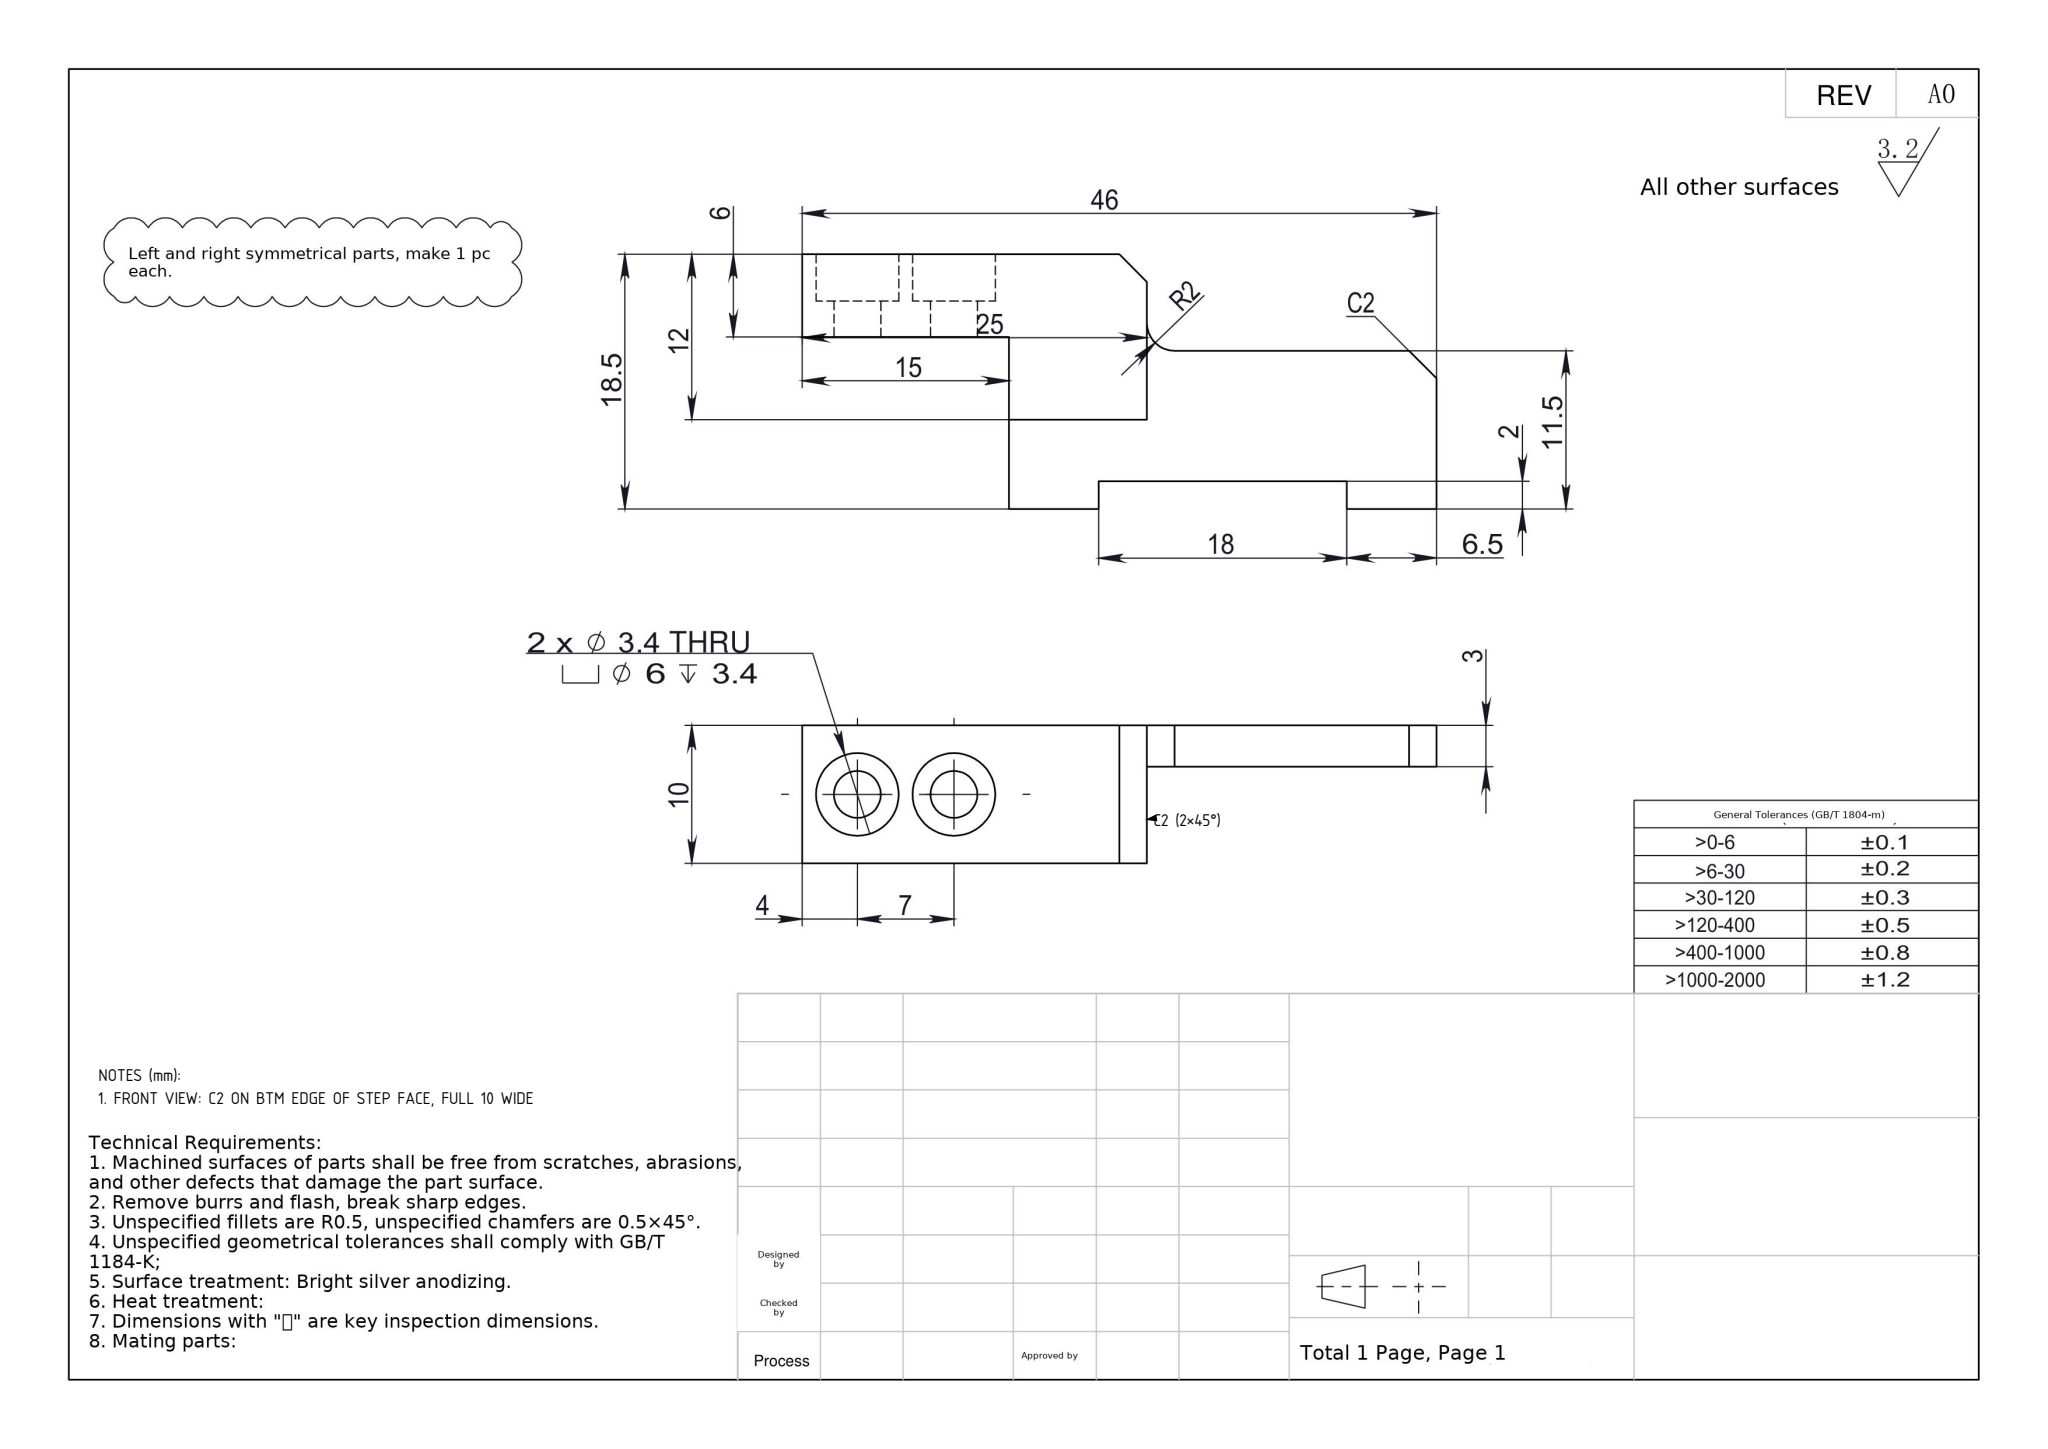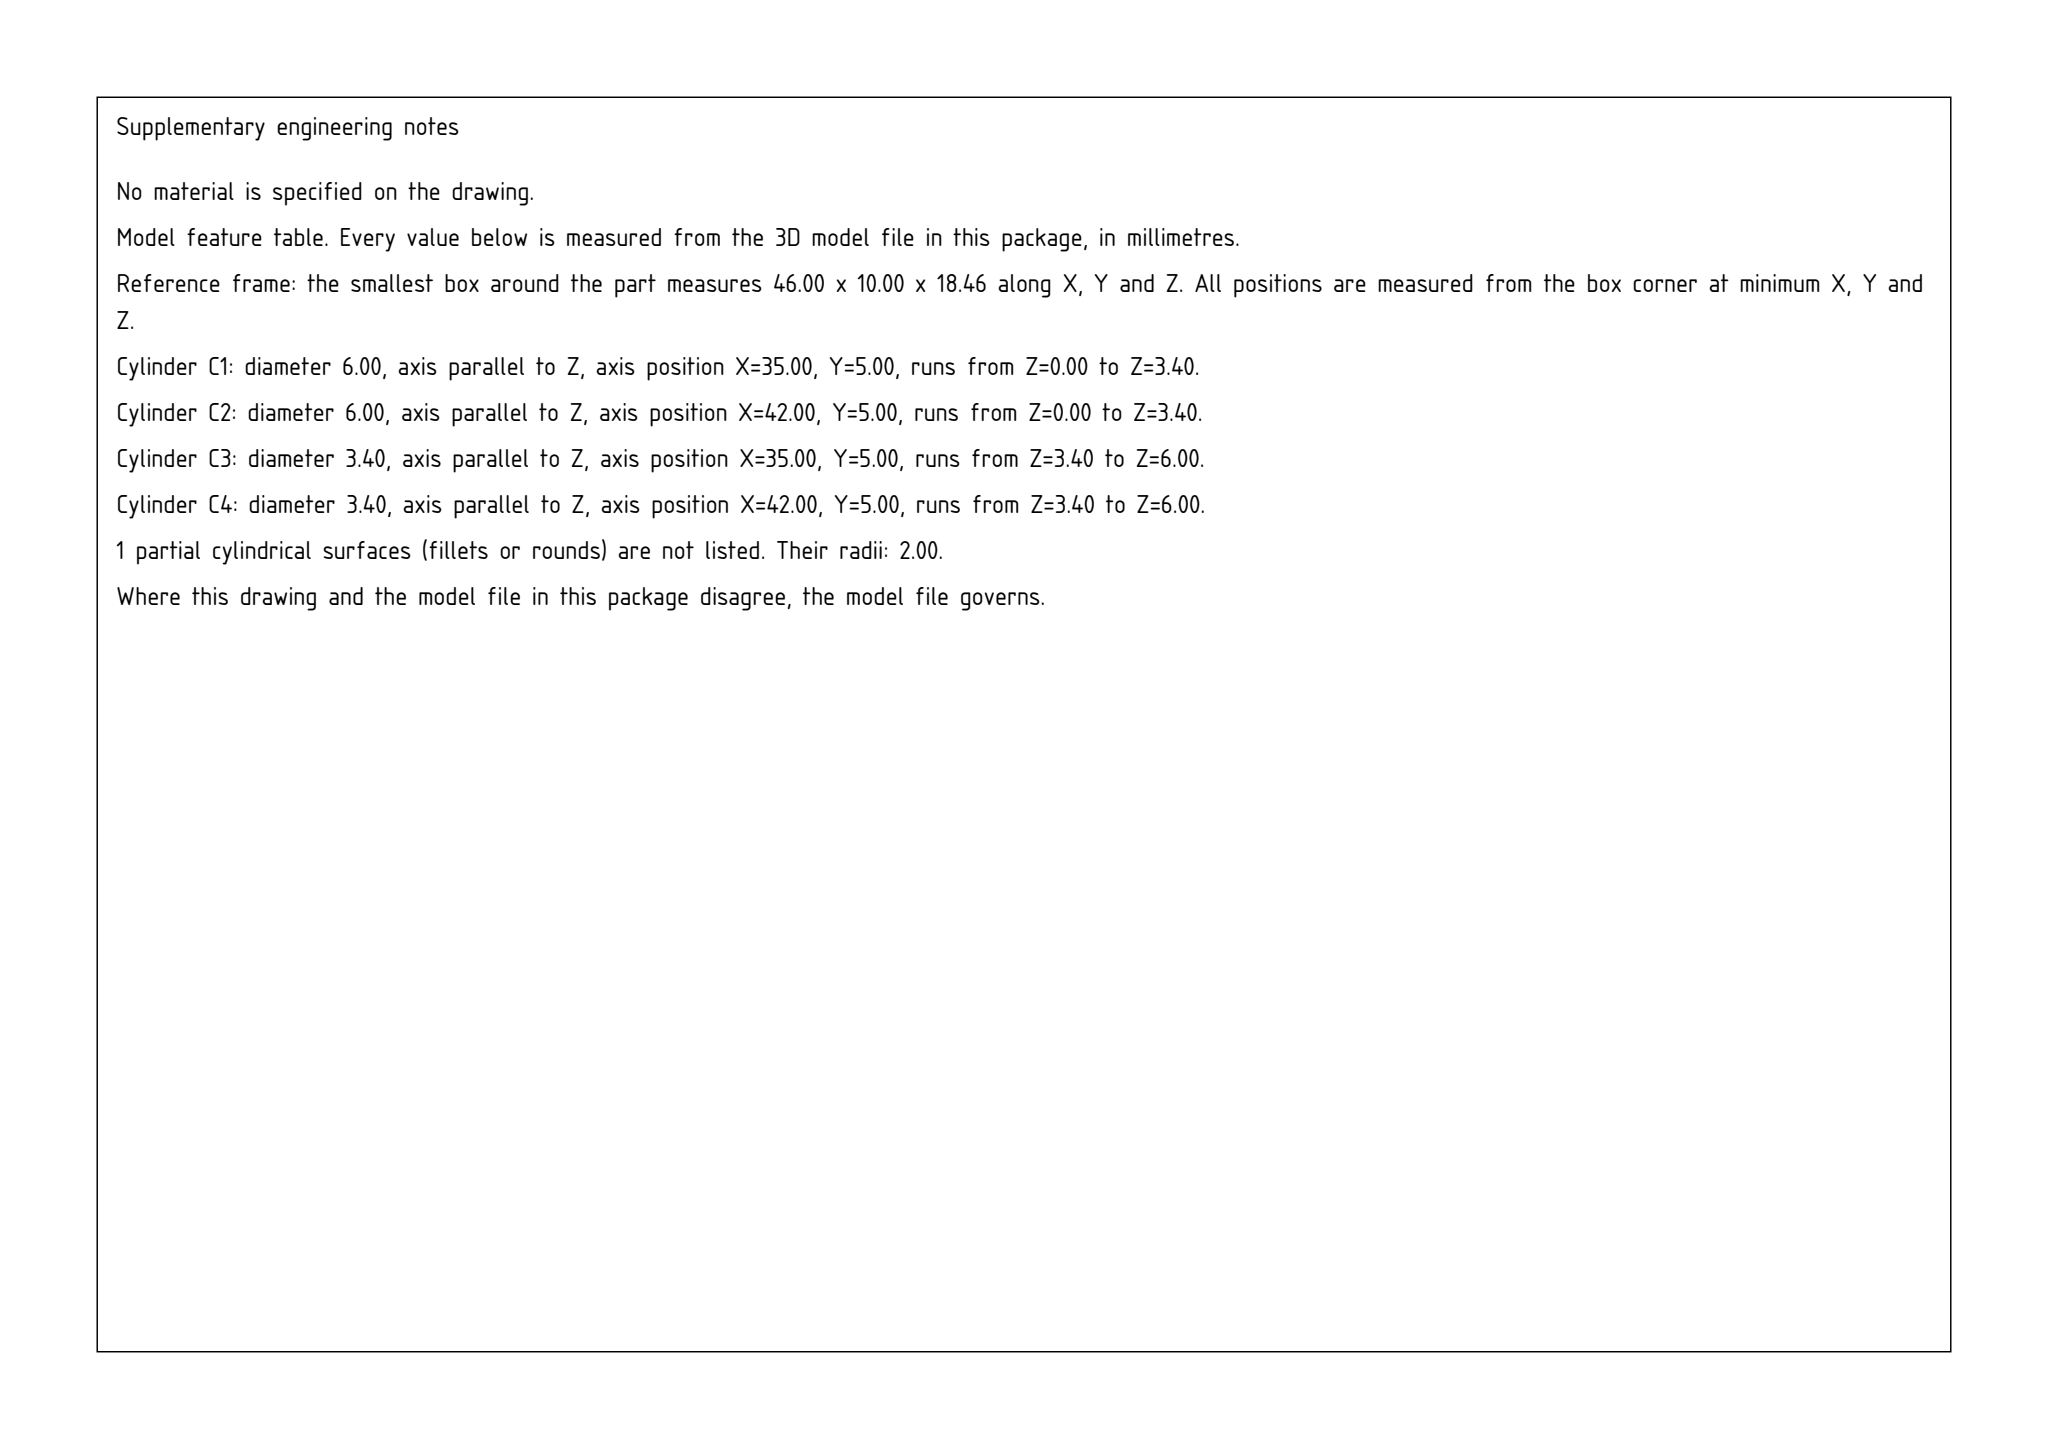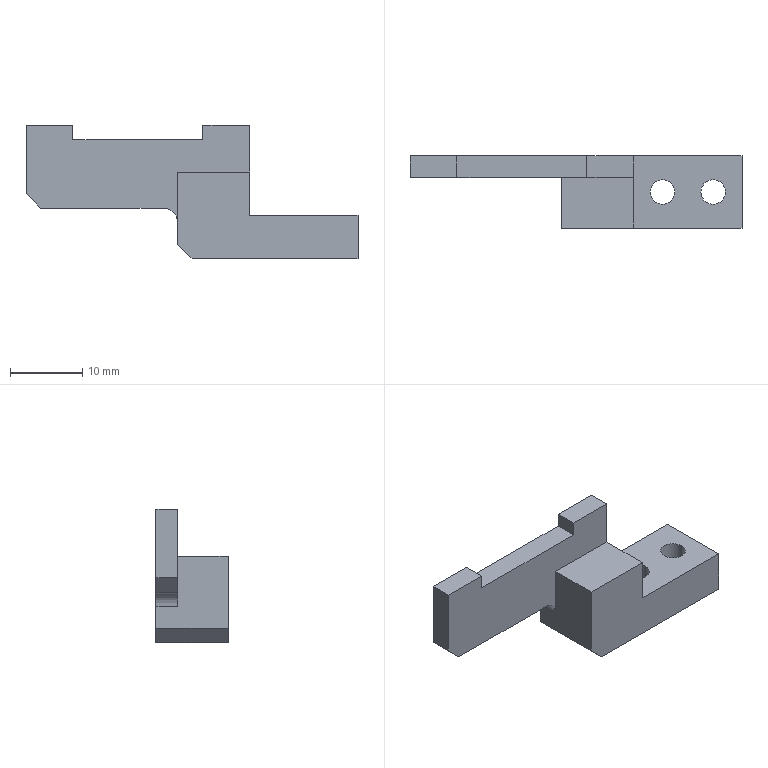Part | SolidWorks | mm | 1 solid | 29 faces | box 46 x 10 x 18.46 mm | volume 2645 mm3 | plane 20 | cylinder 9 | commonest cylinder face diameters 6 x4 3.4 x4 4 x1
Drawing notes:
FRONT VIEW: C2 ON BTM EDGE OF STEP FACE, FULL 10 WIDE | from the solid: inclined plane 45°, bbox_from [21,0,0], size [2,10,2] joining z=0 face and x=21 step face
FRONT VIEW: C2 (2x45 DEG) AT BOTTOM EDGE OF 18 STEP WALL | from the solid: inclined_plane 45/90/45 at bbox_from [21,0,0], size [2,10,2]: 2x2 chamfer between z=0 face (x 23-46) and x=21 face (z from 2)
STEP:
#1=CARTESIAN_POINT('',(-13.,5.,-18.6));
#2=VERTEX_POINT('',#1);
#3=CARTESIAN_POINT('',(-19.,5.,-18.6));
#4=VERTEX_POINT('',#3);
#5=CARTESIAN_POINT('',(-16.,5.,-18.6));
#6=DIRECTION('',(0.,0.,-1.));
#7=DIRECTION('',(-1.,0.,0.));
#8=AXIS2_PLACEMENT_3D('',#5,#6,#7);
#9=CIRCLE('',#8,3.);
#10=EDGE_CURVE('',#2,#4,#9,.T.);
#11=ORIENTED_EDGE('',*,*,#10,.F.);
#12=CARTESIAN_POINT('',(-13.,5.,-22.));
#13=VERTEX_POINT('',#12);
#14=CARTESIAN_POINT('',(-13.,5.,-22.));
#15=DIRECTION('',(0.,0.,-1.));
#16=VECTOR('',#15,1000.);
#17=LINE('',#14,#16);
#18=EDGE_CURVE('',#2,#13,#17,.T.);
#19=ORIENTED_EDGE('',*,*,#18,.T.);
#20=CARTESIAN_POINT('',(-19.,5.,-22.));
#21=VERTEX_POINT('',#20);
#22=CARTESIAN_POINT('',(-16.,5.,-22.));
#23=DIRECTION('',(0.,0.,-1.));
#24=DIRECTION('',(-1.,0.,0.));
#25=AXIS2_PLACEMENT_3D('',#22,#23,#24);
#26=CIRCLE('',#25,3.);
#27=EDGE_CURVE('',#13,#21,#26,.T.);
#28=ORIENTED_EDGE('',*,*,#27,.T.);
#29=CARTESIAN_POINT('',(-19.,5.,-22.));
#30=DIRECTION('',(0.,0.,-1.));
#31=VECTOR('',#30,1000.);
#32=LINE('',#29,#31);
#33=EDGE_CURVE('',#4,#21,#32,.T.);
#34=ORIENTED_EDGE('',*,*,#33,.F.);
#35=EDGE_LOOP('',(#11,#19,#28,#34));
#36=FACE_OUTER_BOUND('',#35,.T.);
#37=CARTESIAN_POINT('',(-16.,5.,-22.));
#38=DIRECTION('',(0.,0.,-1.));
#39=DIRECTION('',(-1.,0.,0.));
#40=AXIS2_PLACEMENT_3D('',#37,#38,#39);
#41=CYLINDRICAL_SURFACE('',#40,3.);
#42=ADVANCED_FACE('',(#36),#41,.F.);
#43=CARTESIAN_POINT('',(-14.3,5.,-16.));
#44=VERTEX_POINT('',#43);
#45=CARTESIAN_POINT('',(-17.7,5.,-16.));
#46=VERTEX_POINT('',#45);
#47=CARTESIAN_POINT('',(-16.,5.,-16.));
#48=DIRECTION('',(-0.,0.,-1.));
#49=DIRECTION('',(-1.,0.,0.));
#50=AXIS2_PLACEMENT_3D('',#47,#48,#49);
#51=CIRCLE('',#50,1.7);
#52=EDGE_CURVE('',#44,#46,#51,.T.);
#53=ORIENTED_EDGE('',*,*,#52,.F.);
#54=CARTESIAN_POINT('',(-14.3,5.,-18.6));
#55=VERTEX_POINT('',#54);
#56=CARTESIAN_POINT('',(-14.3,5.,-22.));
#57=DIRECTION('',(0.,0.,-1.));
#58=VECTOR('',#57,1000.);
#59=LINE('',#56,#58);
#60=EDGE_CURVE('',#44,#55,#59,.T.);
#61=ORIENTED_EDGE('',*,*,#60,.T.);
#62=CARTESIAN_POINT('',(-17.7,5.,-18.6));
#63=VERTEX_POINT('',#62);
#64=CARTESIAN_POINT('',(-16.,5.,-18.6));
#65=DIRECTION('',(0.,0.,-1.));
#66=DIRECTION('',(-1.,0.,0.));
#67=AXIS2_PLACEMENT_3D('',#64,#65,#66);
#68=CIRCLE('',#67,1.7);
#69=EDGE_CURVE('',#55,#63,#68,.T.);
#70=ORIENTED_EDGE('',*,*,#69,.T.);
#71=CARTESIAN_POINT('',(-17.7,5.,-22.));
#72=DIRECTION('',(0.,0.,-1.));
#73=VECTOR('',#72,1000.);
#74=LINE('',#71,#73);
#75=EDGE_CURVE('',#46,#63,#74,.T.);
#76=ORIENTED_EDGE('',*,*,#75,.F.);
#77=EDGE_LOOP('',(#53,#61,#70,#76));
#78=FACE_OUTER_BOUND('',#77,.T.);
#79=CARTESIAN_POINT('',(-16.,5.,-22.));
#80=DIRECTION('',(0.,0.,-1.));
#81=DIRECTION('',(-1.,0.,0.));
#82=AXIS2_PLACEMENT_3D('',#79,#80,#81);
#83=CYLINDRICAL_SURFACE('',#82,1.7);
#84=ADVANCED_FACE('',(#78),#83,.F.);
#85=CARTESIAN_POINT('',(-6.,5.,-18.6));
#86=VERTEX_POINT('',#85);
#87=CARTESIAN_POINT('',(-12.,5.,-18.6));
#88=VERTEX_POINT('',#87);
#89=CARTESIAN_POINT('',(-9.,5.,-18.6));
#90=DIRECTION('',(0.,0.,-1.));
#91=DIRECTION('',(-1.,0.,0.));
#92=AXIS2_PLACEMENT_3D('',#89,#90,#91);
#93=CIRCLE('',#92,3.);
#94=EDGE_CURVE('',#86,#88,#93,.T.);
#95=ORIENTED_EDGE('',*,*,#94,.F.);
#96=CARTESIAN_POINT('',(-6.,5.,-22.));
#97=VERTEX_POINT('',#96);
#98=CARTESIAN_POINT('',(-6.,5.,-22.));
#99=DIRECTION('',(0.,0.,-1.));
#100=VECTOR('',#99,1000.);
#101=LINE('',#98,#100);
#102=EDGE_CURVE('',#86,#97,#101,.T.);
#103=ORIENTED_EDGE('',*,*,#102,.T.);
#104=CARTESIAN_POINT('',(-12.,5.,-22.));
#105=VERTEX_POINT('',#104);
#106=CARTESIAN_POINT('',(-9.,5.,-22.));
#107=DIRECTION('',(0.,0.,-1.));
#108=DIRECTION('',(-1.,0.,0.));
#109=AXIS2_PLACEMENT_3D('',#106,#107,#108);
#110=CIRCLE('',#109,3.);
#111=EDGE_CURVE('',#97,#105,#110,.T.);
#112=ORIENTED_EDGE('',*,*,#111,.T.);
#113=CARTESIAN_POINT('',(-12.,5.,-22.));
#114=DIRECTION('',(0.,0.,-1.));
#115=VECTOR('',#114,1000.);
#116=LINE('',#113,#115);
#117=EDGE_CURVE('',#88,#105,#116,.T.);
#118=ORIENTED_EDGE('',*,*,#117,.F.);
#119=EDGE_LOOP('',(#95,#103,#112,#118));
#120=FACE_OUTER_BOUND('',#119,.T.);
#121=CARTESIAN_POINT('',(-9.,5.,-22.));
#122=DIRECTION('',(0.,0.,-1.));
#123=DIRECTION('',(-1.,0.,0.));
#124=AXIS2_PLACEMENT_3D('',#121,#122,#123);
#125=CYLINDRICAL_SURFACE('',#124,3.);
#126=ADVANCED_FACE('',(#120),#125,.F.);
#127=CARTESIAN_POINT('',(-7.3,5.,-16.));
#128=VERTEX_POINT('',#127);
#129=CARTESIAN_POINT('',(-10.7,5.,-16.));
#130=VERTEX_POINT('',#129);
#131=CARTESIAN_POINT('',(-9.,5.,-16.));
#132=DIRECTION('',(-0.,0.,-1.));
#133=DIRECTION('',(-1.,0.,0.));
#134=AXIS2_PLACEMENT_3D('',#131,#132,#133);
#135=CIRCLE('',#134,1.7);
#136=EDGE_CURVE('',#128,#130,#135,.T.);
#137=ORIENTED_EDGE('',*,*,#136,.F.);
#138=CARTESIAN_POINT('',(-7.3,5.,-18.6));
#139=VERTEX_POINT('',#138);
#140=CARTESIAN_POINT('',(-7.3,5.,-22.));
#141=DIRECTION('',(0.,0.,-1.));
#142=VECTOR('',#141,1000.);
#143=LINE('',#140,#142);
#144=EDGE_CURVE('',#128,#139,#143,.T.);
#145=ORIENTED_EDGE('',*,*,#144,.T.);
#146=CARTESIAN_POINT('',(-10.7,5.,-18.6));
#147=VERTEX_POINT('',#146);
#148=CARTESIAN_POINT('',(-9.,5.,-18.6));
#149=DIRECTION('',(0.,0.,-1.));
#150=DIRECTION('',(-1.,0.,0.));
#151=AXIS2_PLACEMENT_3D('',#148,#149,#150);
#152=CIRCLE('',#151,1.7);
#153=EDGE_CURVE('',#139,#147,#152,.T.);
#154=ORIENTED_EDGE('',*,*,#153,.T.);
#155=CARTESIAN_POINT('',(-10.7,5.,-22.));
#156=DIRECTION('',(0.,0.,-1.));
#157=VECTOR('',#156,1000.);
#158=LINE('',#155,#157);
#159=EDGE_CURVE('',#130,#147,#158,.T.);
#160=ORIENTED_EDGE('',*,*,#159,.F.);
#161=EDGE_LOOP('',(#137,#145,#154,#160));
#162=FACE_OUTER_BOUND('',#161,.T.);
#163=CARTESIAN_POINT('',(-9.,5.,-22.));
#164=DIRECTION('',(0.,0.,-1.));
#165=DIRECTION('',(-1.,0.,0.));
#166=AXIS2_PLACEMENT_3D('',#163,#164,#165);
#167=CYLINDRICAL_SURFACE('',#166,1.7);
#168=ADVANCED_FACE('',(#162),#167,.F.);
#169=CARTESIAN_POINT('',(-44.5,7.,-3.54));
#170=VERTEX_POINT('',#169);
#171=CARTESIAN_POINT('',(-51.,7.,-3.54));
#172=VERTEX_POINT('',#171);
#173=CARTESIAN_POINT('',(-30.,7.,-3.54));
#174=DIRECTION('',(-1.,0.,0.));
#175=VECTOR('',#174,1000.);
#176=LINE('',#173,#175);
#177=EDGE_CURVE('',#170,#172,#176,.T.);
#178=ORIENTED_EDGE('',*,*,#177,.F.);
#179=CARTESIAN_POINT('',(-44.5,10.,-3.54));
#180=VERTEX_POINT('',#179);
#181=CARTESIAN_POINT('',(-44.5,0.,-3.54));
#182=DIRECTION('',(0.,1.,0.));
#183=VECTOR('',#182,1000.);
#184=LINE('',#181,#183);
#185=EDGE_CURVE('',#170,#180,#184,.T.);
#186=ORIENTED_EDGE('',*,*,#185,.T.);
#187=CARTESIAN_POINT('',(-51.,10.,-3.54));
#188=VERTEX_POINT('',#187);
#189=CARTESIAN_POINT('',(-51.762,10.,-3.54));
#190=DIRECTION('',(-1.,0.,0.));
#191=VECTOR('',#190,1000.);
#192=LINE('',#189,#191);
#193=EDGE_CURVE('',#180,#188,#192,.T.);
#194=ORIENTED_EDGE('',*,*,#193,.T.);
#195=CARTESIAN_POINT('',(-51.,10.,-3.54));
#196=DIRECTION('',(0.,1.,0.));
#197=VECTOR('',#196,1000.);
#198=LINE('',#195,#197);
#199=EDGE_CURVE('',#172,#188,#198,.T.);
#200=ORIENTED_EDGE('',*,*,#199,.F.);
#201=EDGE_LOOP('',(#178,#186,#194,#200));
#202=FACE_OUTER_BOUND('',#201,.T.);
#203=CARTESIAN_POINT('',(-51.762,0.,-3.54));
#204=DIRECTION('',(0.,0.,-1.));
#205=DIRECTION('',(-1.,0.,0.));
#206=AXIS2_PLACEMENT_3D('',#203,#204,#205);
#207=PLANE('',#206);
#208=ADVANCED_FACE('',(#202),#207,.F.);
#209=CARTESIAN_POINT('',(-30.,7.,-17.));
#210=VERTEX_POINT('',#209);
#211=CARTESIAN_POINT('',(-30.,7.,-10.));
#212=VERTEX_POINT('',#211);
#213=CARTESIAN_POINT('',(-30.,7.,-15.));
#214=DIRECTION('',(0.,0.,1.));
#215=VECTOR('',#214,1000.);
#216=LINE('',#213,#215);
#217=EDGE_CURVE('',#210,#212,#216,.T.);
#218=ORIENTED_EDGE('',*,*,#217,.F.);
#219=CARTESIAN_POINT('',(-30.,10.,-17.));
#220=VERTEX_POINT('',#219);
#221=CARTESIAN_POINT('',(-30.,0.,-17.));
#222=DIRECTION('',(0.,1.,0.));
#223=VECTOR('',#222,1000.);
#224=LINE('',#221,#223);
#225=EDGE_CURVE('',#210,#220,#224,.T.);
#226=ORIENTED_EDGE('',*,*,#225,.T.);
#227=CARTESIAN_POINT('',(-30.,10.,-20.));
#228=VERTEX_POINT('',#227);
#229=CARTESIAN_POINT('',(-30.,10.,-22.));
#230=DIRECTION('',(0.,0.,-1.));
#231=VECTOR('',#230,1000.);
#232=LINE('',#229,#231);
#233=EDGE_CURVE('',#220,#228,#232,.T.);
#234=ORIENTED_EDGE('',*,*,#233,.T.);
#235=CARTESIAN_POINT('',(-30.,0.,-20.));
#236=VERTEX_POINT('',#235);
#237=CARTESIAN_POINT('',(-30.,0.,-20.));
#238=DIRECTION('',(0.,-1.,0.));
#239=VECTOR('',#238,1000.);
#240=LINE('',#237,#239);
#241=EDGE_CURVE('',#228,#236,#240,.T.);
#242=ORIENTED_EDGE('',*,*,#241,.T.);
#243=CARTESIAN_POINT('',(-30.,0.,-10.));
#244=VERTEX_POINT('',#243);
#245=CARTESIAN_POINT('',(-30.,0.,-22.));
#246=DIRECTION('',(0.,0.,-1.));
#247=VECTOR('',#246,1000.);
#248=LINE('',#245,#247);
#249=EDGE_CURVE('',#244,#236,#248,.T.);
#250=ORIENTED_EDGE('',*,*,#249,.F.);
#251=CARTESIAN_POINT('',(-30.,0.,-10.));
#252=DIRECTION('',(0.,1.,0.));
#253=VECTOR('',#252,1000.);
#254=LINE('',#251,#253);
#255=EDGE_CURVE('',#244,#212,#254,.T.);
#256=ORIENTED_EDGE('',*,*,#255,.T.);
#257=EDGE_LOOP('',(#218,#226,#234,#242,#250,#256));
#258=FACE_OUTER_BOUND('',#257,.T.);
#259=CARTESIAN_POINT('',(-30.,0.,-22.));
#260=DIRECTION('',(1.,0.,0.));
#261=DIRECTION('',(0.,0.,-1.));
#262=AXIS2_PLACEMENT_3D('',#259,#260,#261);
#263=PLANE('',#262);
#264=ADVANCED_FACE('',(#258),#263,.F.);
#265=CARTESIAN_POINT('',(-16.,5.,-22.));
#266=DIRECTION('',(0.,0.,-1.));
#267=DIRECTION('',(-1.,0.,0.));
#268=AXIS2_PLACEMENT_3D('',#265,#266,#267);
#269=CIRCLE('',#268,3.);
#270=EDGE_CURVE('',#21,#13,#269,.T.);
#271=ORIENTED_EDGE('',*,*,#270,.F.);
#272=ORIENTED_EDGE('',*,*,#27,.F.);
#273=EDGE_LOOP('',(#271,#272));
#274=FACE_BOUND('',#273,.T.);
#275=CARTESIAN_POINT('',(-9.,5.,-22.));
#276=DIRECTION('',(0.,0.,-1.));
#277=DIRECTION('',(-1.,0.,0.));
#278=AXIS2_PLACEMENT_3D('',#275,#276,#277);
#279=CIRCLE('',#278,3.);
#280=EDGE_CURVE('',#105,#97,#279,.T.);
#281=ORIENTED_EDGE('',*,*,#280,.F.);
#282=ORIENTED_EDGE('',*,*,#111,.F.);
#283=EDGE_LOOP('',(#281,#282));
#284=FACE_BOUND('',#283,.T.);
#285=CARTESIAN_POINT('',(-5.,10.,-22.));
#286=VERTEX_POINT('',#285);
#287=CARTESIAN_POINT('',(-28.,10.,-22.));
#288=VERTEX_POINT('',#287);
#289=CARTESIAN_POINT('',(0.,10.,-22.));
#290=DIRECTION('',(-1.,0.,0.));
#291=VECTOR('',#290,1000.);
#292=LINE('',#289,#291);
#293=EDGE_CURVE('',#286,#288,#292,.T.);
#294=ORIENTED_EDGE('',*,*,#293,.F.);
#295=CARTESIAN_POINT('',(-5.,0.,-22.));
#296=VERTEX_POINT('',#295);
#297=CARTESIAN_POINT('',(-5.,22.249,-22.));
#298=DIRECTION('',(0.,1.,0.));
#299=VECTOR('',#298,1000.);
#300=LINE('',#297,#299);
#301=EDGE_CURVE('',#296,#286,#300,.T.);
#302=ORIENTED_EDGE('',*,*,#301,.F.);
#303=CARTESIAN_POINT('',(-28.,0.,-22.));
#304=VERTEX_POINT('',#303);
#305=CARTESIAN_POINT('',(0.,0.,-22.));
#306=DIRECTION('',(-1.,0.,0.));
#307=VECTOR('',#306,1000.);
#308=LINE('',#305,#307);
#309=EDGE_CURVE('',#296,#304,#308,.T.);
#310=ORIENTED_EDGE('',*,*,#309,.T.);
#311=CARTESIAN_POINT('',(-28.,10.,-22.));
#312=DIRECTION('',(0.,1.,0.));
#313=VECTOR('',#312,1000.);
#314=LINE('',#311,#313);
#315=EDGE_CURVE('',#304,#288,#314,.T.);
#316=ORIENTED_EDGE('',*,*,#315,.T.);
#317=EDGE_LOOP('',(#294,#302,#310,#316));
#318=FACE_OUTER_BOUND('',#317,.T.);
#319=CARTESIAN_POINT('',(0.,10.,-22.));
#320=DIRECTION('',(0.,0.,1.));
#321=DIRECTION('',(1.,0.,-0.));
#322=AXIS2_PLACEMENT_3D('',#319,#320,#321);
#323=PLANE('',#322);
#324=ADVANCED_FACE('',(#274,#284,#318),#323,.F.);
#325=CARTESIAN_POINT('',(-44.5,10.,-5.54));
#326=VERTEX_POINT('',#325);
#327=CARTESIAN_POINT('',(-44.5,10.,-1.54));
#328=DIRECTION('',(0.,0.,-1.));
#329=VECTOR('',#328,1000.);
#330=LINE('',#327,#329);
#331=EDGE_CURVE('',#180,#326,#330,.T.);
#332=ORIENTED_EDGE('',*,*,#331,.T.);
#333=CARTESIAN_POINT('',(-26.5,10.,-5.54));
#334=VERTEX_POINT('',#333);
#335=CARTESIAN_POINT('',(-26.5,10.,-5.54));
#336=DIRECTION('',(1.,0.,-0.));
#337=VECTOR('',#336,1000.);
#338=LINE('',#335,#337);
#339=EDGE_CURVE('',#326,#334,#338,.T.);
#340=ORIENTED_EDGE('',*,*,#339,.T.);
#341=CARTESIAN_POINT('',(-26.5,10.,-3.54));
#342=VERTEX_POINT('',#341);
#343=CARTESIAN_POINT('',(-26.5,10.,-1.54));
#344=DIRECTION('',(0.,0.,1.));
#345=VECTOR('',#344,1000.);
#346=LINE('',#343,#345);
#347=EDGE_CURVE('',#334,#342,#346,.T.);
#348=ORIENTED_EDGE('',*,*,#347,.T.);
#349=CARTESIAN_POINT('',(-20.,10.,-3.54));
#350=VERTEX_POINT('',#349);
#351=CARTESIAN_POINT('',(-51.762,10.,-3.54));
#352=DIRECTION('',(-1.,0.,0.));
#353=VECTOR('',#352,1000.);
#354=LINE('',#351,#353);
#355=EDGE_CURVE('',#350,#342,#354,.T.);
#356=ORIENTED_EDGE('',*,*,#355,.F.);
#357=CARTESIAN_POINT('',(-20.,10.,-16.));
#358=VERTEX_POINT('',#357);
#359=CARTESIAN_POINT('',(-20.,10.,0.));
#360=DIRECTION('',(0.,0.,1.));
#361=VECTOR('',#360,1000.);
#362=LINE('',#359,#361);
#363=EDGE_CURVE('',#358,#350,#362,.T.);
#364=ORIENTED_EDGE('',*,*,#363,.F.);
#365=CARTESIAN_POINT('',(-5.,10.,-16.));
#366=VERTEX_POINT('',#365);
#367=CARTESIAN_POINT('',(0.,10.,-16.));
#368=DIRECTION('',(-1.,0.,0.));
#369=VECTOR('',#368,1000.);
#370=LINE('',#367,#369);
#371=EDGE_CURVE('',#366,#358,#370,.T.);
#372=ORIENTED_EDGE('',*,*,#371,.F.);
#373=CARTESIAN_POINT('',(-5.,10.,0.));
#374=DIRECTION('',(0.,0.,1.));
#375=VECTOR('',#374,1000.);
#376=LINE('',#373,#375);
#377=EDGE_CURVE('',#286,#366,#376,.T.);
#378=ORIENTED_EDGE('',*,*,#377,.F.);
#379=ORIENTED_EDGE('',*,*,#293,.T.);
#380=CARTESIAN_POINT('',(-25.,10.,-25.));
#381=DIRECTION('',(-0.7071,0.,0.7071));
#382=VECTOR('',#381,1000.);
#383=LINE('',#380,#382);
#384=EDGE_CURVE('',#288,#228,#383,.T.);
#385=ORIENTED_EDGE('',*,*,#384,.T.);
#386=ORIENTED_EDGE('',*,*,#233,.F.);
#387=CARTESIAN_POINT('',(-32.,10.,-15.));
#388=VERTEX_POINT('',#387);
#389=CARTESIAN_POINT('',(-32.,10.,-17.));
#390=DIRECTION('',(0.,-1.,0.));
#391=DIRECTION('',(0.,0.,1.));
#392=AXIS2_PLACEMENT_3D('',#389,#390,#391);
#393=CIRCLE('',#392,2.);
#394=EDGE_CURVE('',#220,#388,#393,.T.);
#395=ORIENTED_EDGE('',*,*,#394,.T.);
#396=CARTESIAN_POINT('',(-49.,10.,-15.));
#397=VERTEX_POINT('',#396);
#398=CARTESIAN_POINT('',(-51.,10.,-15.));
#399=DIRECTION('',(1.,0.,0.));
#400=VECTOR('',#399,1000.);
#401=LINE('',#398,#400);
#402=EDGE_CURVE('',#397,#388,#401,.T.);
#403=ORIENTED_EDGE('',*,*,#402,.F.);
#404=CARTESIAN_POINT('',(-51.,10.,-13.));
#405=VERTEX_POINT('',#404);
#406=CARTESIAN_POINT('',(-32.,10.,-32.));
#407=DIRECTION('',(-0.7071,0.,0.7071));
#408=VECTOR('',#407,1000.);
#409=LINE('',#406,#408);
#410=EDGE_CURVE('',#397,#405,#409,.T.);
#411=ORIENTED_EDGE('',*,*,#410,.T.);
#412=CARTESIAN_POINT('',(-51.,10.,11.14));
#413=DIRECTION('',(-0.,0.,1.));
#414=VECTOR('',#413,1000.);
#415=LINE('',#412,#414);
#416=EDGE_CURVE('',#405,#188,#415,.T.);
#417=ORIENTED_EDGE('',*,*,#416,.T.);
#418=ORIENTED_EDGE('',*,*,#193,.F.);
#419=EDGE_LOOP('',(#332,#340,#348,#356,#364,#372,#378,#379,#385,#386,#395,#403,#411,#417,#418));
#420=FACE_OUTER_BOUND('',#419,.T.);
#421=CARTESIAN_POINT('',(0.,10.,0.));
#422=DIRECTION('',(0.,1.,0.));
#423=DIRECTION('',(0.,0.,1.));
#424=AXIS2_PLACEMENT_3D('',#421,#422,#423);
#425=PLANE('',#424);
#426=ADVANCED_FACE('',(#420),#425,.T.);
#427=ORIENTED_EDGE('',*,*,#309,.F.);
#428=CARTESIAN_POINT('',(-5.,0.,-16.));
#429=VERTEX_POINT('',#428);
#430=CARTESIAN_POINT('',(-5.,0.,0.));
#431=DIRECTION('',(0.,0.,1.));
#432=VECTOR('',#431,1000.);
#433=LINE('',#430,#432);
#434=EDGE_CURVE('',#296,#429,#433,.T.);
#435=ORIENTED_EDGE('',*,*,#434,.T.);
#436=CARTESIAN_POINT('',(-20.,0.,-16.));
#437=VERTEX_POINT('',#436);
#438=CARTESIAN_POINT('',(0.,0.,-16.));
#439=DIRECTION('',(-1.,0.,0.));
#440=VECTOR('',#439,1000.);
#441=LINE('',#438,#440);
#442=EDGE_CURVE('',#429,#437,#441,.T.);
#443=ORIENTED_EDGE('',*,*,#442,.T.);
#444=CARTESIAN_POINT('',(-20.,0.,-10.));
#445=VERTEX_POINT('',#444);
#446=CARTESIAN_POINT('',(-20.,0.,0.));
#447=DIRECTION('',(0.,0.,1.));
#448=VECTOR('',#447,1000.);
#449=LINE('',#446,#448);
#450=EDGE_CURVE('',#437,#445,#449,.T.);
#451=ORIENTED_EDGE('',*,*,#450,.T.);
#452=CARTESIAN_POINT('',(-20.,0.,-10.));
#453=DIRECTION('',(1.,0.,0.));
#454=VECTOR('',#453,1000.);
#455=LINE('',#452,#454);
#456=EDGE_CURVE('',#244,#445,#455,.T.);
#457=ORIENTED_EDGE('',*,*,#456,.F.);
#458=ORIENTED_EDGE('',*,*,#249,.T.);
#459=CARTESIAN_POINT('',(-28.,0.,-22.));
#460=DIRECTION('',(0.7071,0.,-0.7071));
#461=VECTOR('',#460,1000.);
#462=LINE('',#459,#461);
#463=EDGE_CURVE('',#236,#304,#462,.T.);
#464=ORIENTED_EDGE('',*,*,#463,.T.);
#465=EDGE_LOOP('',(#427,#435,#443,#451,#457,#458,#464));
#466=FACE_OUTER_BOUND('',#465,.T.);
#467=CARTESIAN_POINT('',(0.,0.,0.));
#468=DIRECTION('',(0.,1.,0.));
#469=DIRECTION('',(0.,0.,1.));
#470=AXIS2_PLACEMENT_3D('',#467,#468,#469);
#471=PLANE('',#470);
#472=ADVANCED_FACE('',(#466),#471,.F.);
#473=ORIENTED_EDGE('',*,*,#363,.T.);
#474=CARTESIAN_POINT('',(-20.,7.,-3.54));
#475=VERTEX_POINT('',#474);
#476=CARTESIAN_POINT('',(-20.,0.,-3.54));
#477=DIRECTION('',(0.,-1.,0.));
#478=VECTOR('',#477,1000.);
#479=LINE('',#476,#478);
#480=EDGE_CURVE('',#350,#475,#479,.T.);
#481=ORIENTED_EDGE('',*,*,#480,.T.);
#482=CARTESIAN_POINT('',(-20.,7.,-10.));
#483=VERTEX_POINT('',#482);
#484=CARTESIAN_POINT('',(-20.,7.,0.));
#485=DIRECTION('',(0.,0.,1.));
#486=VECTOR('',#485,1000.);
#487=LINE('',#484,#486);
#488=EDGE_CURVE('',#483,#475,#487,.T.);
#489=ORIENTED_EDGE('',*,*,#488,.F.);
#490=CARTESIAN_POINT('',(-20.,27.435,-10.));
#491=DIRECTION('',(0.,-1.,0.));
#492=VECTOR('',#491,1000.);
#493=LINE('',#490,#492);
#494=EDGE_CURVE('',#483,#445,#493,.T.);
#495=ORIENTED_EDGE('',*,*,#494,.T.);
#496=ORIENTED_EDGE('',*,*,#450,.F.);
#497=CARTESIAN_POINT('',(-20.,0.,-16.));
#498=DIRECTION('',(0.,1.,0.));
#499=VECTOR('',#498,1000.);
#500=LINE('',#497,#499);
#501=EDGE_CURVE('',#437,#358,#500,.T.);
#502=ORIENTED_EDGE('',*,*,#501,.T.);
#503=EDGE_LOOP('',(#473,#481,#489,#495,#496,#502));
#504=FACE_OUTER_BOUND('',#503,.T.);
#505=CARTESIAN_POINT('',(-20.,0.,0.));
#506=DIRECTION('',(-1.,0.,0.));
#507=DIRECTION('',(0.,0.,1.));
#508=AXIS2_PLACEMENT_3D('',#505,#506,#507);
#509=PLANE('',#508);
#510=ADVANCED_FACE('',(#504),#509,.F.);
#511=CARTESIAN_POINT('',(-16.,5.,-16.));
#512=DIRECTION('',(-0.,0.,-1.));
#513=DIRECTION('',(-1.,0.,0.));
#514=AXIS2_PLACEMENT_3D('',#511,#512,#513);
#515=CIRCLE('',#514,1.7);
#516=EDGE_CURVE('',#46,#44,#515,.T.);
#517=ORIENTED_EDGE('',*,*,#516,.T.);
#518=ORIENTED_EDGE('',*,*,#52,.T.);
#519=EDGE_LOOP('',(#517,#518));
#520=FACE_BOUND('',#519,.T.);
#521=CARTESIAN_POINT('',(-9.,5.,-16.));
#522=DIRECTION('',(-0.,0.,-1.));
#523=DIRECTION('',(-1.,0.,0.));
#524=AXIS2_PLACEMENT_3D('',#521,#522,#523);
#525=CIRCLE('',#524,1.7);
#526=EDGE_CURVE('',#130,#128,#525,.T.);
#527=ORIENTED_EDGE('',*,*,#526,.T.);
#528=ORIENTED_EDGE('',*,*,#136,.T.);
#529=EDGE_LOOP('',(#527,#528));
#530=FACE_BOUND('',#529,.T.);
#531=ORIENTED_EDGE('',*,*,#442,.F.);
#532=CARTESIAN_POINT('',(-5.,0.,-16.));
#533=DIRECTION('',(0.,1.,0.));
#534=VECTOR('',#533,1000.);
#535=LINE('',#532,#534);
#536=EDGE_CURVE('',#429,#366,#535,.T.);
#537=ORIENTED_EDGE('',*,*,#536,.T.);
#538=ORIENTED_EDGE('',*,*,#371,.T.);
#539=ORIENTED_EDGE('',*,*,#501,.F.);
#540=EDGE_LOOP('',(#531,#537,#538,#539));
#541=FACE_OUTER_BOUND('',#540,.T.);
#542=CARTESIAN_POINT('',(0.,0.,-16.));
#543=DIRECTION('',(-0.,0.,-1.));
#544=DIRECTION('',(-1.,0.,0.));
#545=AXIS2_PLACEMENT_3D('',#542,#543,#544);
#546=PLANE('',#545);
#547=ADVANCED_FACE('',(#520,#530,#541),#546,.F.);
#548=ORIENTED_EDGE('',*,*,#144,.F.);
#549=ORIENTED_EDGE('',*,*,#526,.F.);
#550=ORIENTED_EDGE('',*,*,#159,.T.);
#551=CARTESIAN_POINT('',(-9.,5.,-18.6));
#552=DIRECTION('',(0.,0.,-1.));
#553=DIRECTION('',(-1.,0.,0.));
#554=AXIS2_PLACEMENT_3D('',#551,#552,#553);
#555=CIRCLE('',#554,1.7);
#556=EDGE_CURVE('',#147,#139,#555,.T.);
#557=ORIENTED_EDGE('',*,*,#556,.T.);
#558=EDGE_LOOP('',(#548,#549,#550,#557));
#559=FACE_OUTER_BOUND('',#558,.T.);
#560=CARTESIAN_POINT('',(-9.,5.,-22.));
#561=DIRECTION('',(0.,0.,-1.));
#562=DIRECTION('',(-1.,0.,0.));
#563=AXIS2_PLACEMENT_3D('',#560,#561,#562);
#564=CYLINDRICAL_SURFACE('',#563,1.7);
#565=ADVANCED_FACE('',(#559),#564,.F.);
#566=ORIENTED_EDGE('',*,*,#556,.F.);
#567=ORIENTED_EDGE('',*,*,#153,.F.);
#568=EDGE_LOOP('',(#566,#567));
#569=FACE_BOUND('',#568,.T.);
#570=CARTESIAN_POINT('',(-9.,5.,-18.6));
#571=DIRECTION('',(0.,0.,-1.));
#572=DIRECTION('',(-1.,0.,0.));
#573=AXIS2_PLACEMENT_3D('',#570,#571,#572);
#574=CIRCLE('',#573,3.);
#575=EDGE_CURVE('',#88,#86,#574,.T.);
#576=ORIENTED_EDGE('',*,*,#575,.T.);
#577=ORIENTED_EDGE('',*,*,#94,.T.);
#578=EDGE_LOOP('',(#576,#577));
#579=FACE_OUTER_BOUND('',#578,.T.);
#580=CARTESIAN_POINT('',(-7.3,5.,-18.6));
#581=DIRECTION('',(0.,0.,1.));
#582=DIRECTION('',(1.,0.,0.));
#583=AXIS2_PLACEMENT_3D('',#580,#581,#582);
#584=PLANE('',#583);
#585=ADVANCED_FACE('',(#569,#579),#584,.F.);
#586=ORIENTED_EDGE('',*,*,#102,.F.);
#587=ORIENTED_EDGE('',*,*,#575,.F.);
#588=ORIENTED_EDGE('',*,*,#117,.T.);
#589=ORIENTED_EDGE('',*,*,#280,.T.);
#590=EDGE_LOOP('',(#586,#587,#588,#589));
#591=FACE_OUTER_BOUND('',#590,.T.);
#592=CARTESIAN_POINT('',(-9.,5.,-22.));
#593=DIRECTION('',(0.,0.,-1.));
#594=DIRECTION('',(-1.,0.,0.));
#595=AXIS2_PLACEMENT_3D('',#592,#593,#594);
#596=CYLINDRICAL_SURFACE('',#595,3.);
#597=ADVANCED_FACE('',(#591),#596,.F.);
#598=ORIENTED_EDGE('',*,*,#60,.F.);
#599=ORIENTED_EDGE('',*,*,#516,.F.);
#600=ORIENTED_EDGE('',*,*,#75,.T.);
#601=CARTESIAN_POINT('',(-16.,5.,-18.6));
#602=DIRECTION('',(0.,0.,-1.));
#603=DIRECTION('',(-1.,0.,0.));
#604=AXIS2_PLACEMENT_3D('',#601,#602,#603);
#605=CIRCLE('',#604,1.7);
#606=EDGE_CURVE('',#63,#55,#605,.T.);
#607=ORIENTED_EDGE('',*,*,#606,.T.);
#608=EDGE_LOOP('',(#598,#599,#600,#607));
#609=FACE_OUTER_BOUND('',#608,.T.);
#610=CARTESIAN_POINT('',(-16.,5.,-22.));
#611=DIRECTION('',(0.,0.,-1.));
#612=DIRECTION('',(-1.,0.,0.));
#613=AXIS2_PLACEMENT_3D('',#610,#611,#612);
#614=CYLINDRICAL_SURFACE('',#613,1.7);
#615=ADVANCED_FACE('',(#609),#614,.F.);
#616=ORIENTED_EDGE('',*,*,#606,.F.);
#617=ORIENTED_EDGE('',*,*,#69,.F.);
#618=EDGE_LOOP('',(#616,#617));
#619=FACE_BOUND('',#618,.T.);
#620=CARTESIAN_POINT('',(-16.,5.,-18.6));
#621=DIRECTION('',(0.,0.,-1.));
#622=DIRECTION('',(-1.,0.,0.));
#623=AXIS2_PLACEMENT_3D('',#620,#621,#622);
#624=CIRCLE('',#623,3.);
#625=EDGE_CURVE('',#4,#2,#624,.T.);
#626=ORIENTED_EDGE('',*,*,#625,.T.);
#627=ORIENTED_EDGE('',*,*,#10,.T.);
#628=EDGE_LOOP('',(#626,#627));
#629=FACE_OUTER_BOUND('',#628,.T.);
#630=CARTESIAN_POINT('',(-14.3,5.,-18.6));
#631=DIRECTION('',(0.,0.,1.));
#632=DIRECTION('',(1.,0.,0.));
#633=AXIS2_PLACEMENT_3D('',#630,#631,#632);
#634=PLANE('',#633);
#635=ADVANCED_FACE('',(#619,#629),#634,.F.);
#636=ORIENTED_EDGE('',*,*,#18,.F.);
#637=ORIENTED_EDGE('',*,*,#625,.F.);
#638=ORIENTED_EDGE('',*,*,#33,.T.);
#639=ORIENTED_EDGE('',*,*,#270,.T.);
#640=EDGE_LOOP('',(#636,#637,#638,#639));
#641=FACE_OUTER_BOUND('',#640,.T.);
#642=CARTESIAN_POINT('',(-16.,5.,-22.));
#643=DIRECTION('',(0.,0.,-1.));
#644=DIRECTION('',(-1.,0.,0.));
#645=AXIS2_PLACEMENT_3D('',#642,#643,#644);
#646=CYLINDRICAL_SURFACE('',#645,3.);
#647=ADVANCED_FACE('',(#641),#646,.F.);
#648=ORIENTED_EDGE('',*,*,#463,.F.);
#649=ORIENTED_EDGE('',*,*,#241,.F.);
#650=ORIENTED_EDGE('',*,*,#384,.F.);
#651=ORIENTED_EDGE('',*,*,#315,.F.);
#652=EDGE_LOOP('',(#648,#649,#650,#651));
#653=FACE_OUTER_BOUND('',#652,.T.);
#654=CARTESIAN_POINT('',(-28.,10.,-22.));
#655=DIRECTION('',(0.7071,0.,0.7071));
#656=DIRECTION('',(0.,1.,0.));
#657=AXIS2_PLACEMENT_3D('',#654,#655,#656);
#658=PLANE('',#657);
#659=ADVANCED_FACE('',(#653),#658,.F.);
#660=CARTESIAN_POINT('',(-44.5,7.,-5.54));
#661=VERTEX_POINT('',#660);
#662=CARTESIAN_POINT('',(-26.5,7.,-5.54));
#663=VERTEX_POINT('',#662);
#664=CARTESIAN_POINT('',(-26.5,7.,-5.54));
#665=DIRECTION('',(1.,0.,-0.));
#666=VECTOR('',#665,1000.);
#667=LINE('',#664,#666);
#668=EDGE_CURVE('',#661,#663,#667,.T.);
#669=ORIENTED_EDGE('',*,*,#668,.F.);
#670=CARTESIAN_POINT('',(-44.5,7.,-1.54));
#671=DIRECTION('',(0.,0.,-1.));
#672=VECTOR('',#671,1000.);
#673=LINE('',#670,#672);
#674=EDGE_CURVE('',#170,#661,#673,.T.);
#675=ORIENTED_EDGE('',*,*,#674,.F.);
#676=ORIENTED_EDGE('',*,*,#177,.T.);
#677=CARTESIAN_POINT('',(-51.,7.,-13.));
#678=VERTEX_POINT('',#677);
#679=CARTESIAN_POINT('',(-51.,7.,11.14));
#680=DIRECTION('',(-0.,0.,1.));
#681=VECTOR('',#680,1000.);
#682=LINE('',#679,#681);
#683=EDGE_CURVE('',#678,#172,#682,.T.);
#684=ORIENTED_EDGE('',*,*,#683,.F.);
#685=CARTESIAN_POINT('',(-49.,7.,-15.));
#686=VERTEX_POINT('',#685);
#687=CARTESIAN_POINT('',(-49.,7.,-15.));
#688=DIRECTION('',(0.7071,0.,-0.7071));
#689=VECTOR('',#688,1000.);
#690=LINE('',#687,#689);
#691=EDGE_CURVE('',#678,#686,#690,.T.);
#692=ORIENTED_EDGE('',*,*,#691,.T.);
#693=CARTESIAN_POINT('',(-32.,7.,-15.));
#694=VERTEX_POINT('',#693);
#695=CARTESIAN_POINT('',(-30.,7.,-15.));
#696=DIRECTION('',(-1.,0.,0.));
#697=VECTOR('',#696,1000.);
#698=LINE('',#695,#697);
#699=EDGE_CURVE('',#694,#686,#698,.T.);
#700=ORIENTED_EDGE('',*,*,#699,.F.);
#701=CARTESIAN_POINT('',(-32.,7.,-17.));
#702=DIRECTION('',(0.,1.,0.));
#703=DIRECTION('',(0.,0.,1.));
#704=AXIS2_PLACEMENT_3D('',#701,#702,#703);
#705=CIRCLE('',#704,2.);
#706=EDGE_CURVE('',#694,#210,#705,.T.);
#707=ORIENTED_EDGE('',*,*,#706,.T.);
#708=ORIENTED_EDGE('',*,*,#217,.T.);
#709=CARTESIAN_POINT('',(-20.,7.,-10.));
#710=DIRECTION('',(1.,0.,0.));
#711=VECTOR('',#710,1000.);
#712=LINE('',#709,#711);
#713=EDGE_CURVE('',#212,#483,#712,.T.);
#714=ORIENTED_EDGE('',*,*,#713,.T.);
#715=ORIENTED_EDGE('',*,*,#488,.T.);
#716=CARTESIAN_POINT('',(-26.5,7.,-3.54));
#717=VERTEX_POINT('',#716);
#718=CARTESIAN_POINT('',(-30.,7.,-3.54));
#719=DIRECTION('',(-1.,0.,0.));
#720=VECTOR('',#719,1000.);
#721=LINE('',#718,#720);
#722=EDGE_CURVE('',#475,#717,#721,.T.);
#723=ORIENTED_EDGE('',*,*,#722,.T.);
#724=CARTESIAN_POINT('',(-26.5,7.,-1.54));
#725=DIRECTION('',(0.,0.,1.));
#726=VECTOR('',#725,1000.);
#727=LINE('',#724,#726);
#728=EDGE_CURVE('',#663,#717,#727,.T.);
#729=ORIENTED_EDGE('',*,*,#728,.F.);
#730=EDGE_LOOP('',(#669,#675,#676,#684,#692,#700,#707,#708,#714,#715,#723,#729));
#731=FACE_OUTER_BOUND('',#730,.T.);
#732=CARTESIAN_POINT('',(-30.,7.,0.));
#733=DIRECTION('',(0.,1.,0.));
#734=DIRECTION('',(0.,0.,1.));
#735=AXIS2_PLACEMENT_3D('',#732,#733,#734);
#736=PLANE('',#735);
#737=ADVANCED_FACE('',(#731),#736,.F.);
#738=ORIENTED_EDGE('',*,*,#416,.F.);
#739=CARTESIAN_POINT('',(-51.,7.,-13.));
#740=DIRECTION('',(0.,-1.,0.));
#741=VECTOR('',#740,1000.);
#742=LINE('',#739,#741);
#743=EDGE_CURVE('',#405,#678,#742,.T.);
#744=ORIENTED_EDGE('',*,*,#743,.T.);
#745=ORIENTED_EDGE('',*,*,#683,.T.);
#746=ORIENTED_EDGE('',*,*,#199,.T.);
#747=EDGE_LOOP('',(#738,#744,#745,#746));
#748=FACE_OUTER_BOUND('',#747,.T.);
#749=CARTESIAN_POINT('',(-51.,10.,11.14));
#750=DIRECTION('',(1.,0.,0.));
#751=DIRECTION('',(0.,0.,-1.));
#752=AXIS2_PLACEMENT_3D('',#749,#750,#751);
#753=PLANE('',#752);
#754=ADVANCED_FACE('',(#748),#753,.F.);
#755=ORIENTED_EDGE('',*,*,#456,.T.);
#756=ORIENTED_EDGE('',*,*,#494,.F.);
#757=ORIENTED_EDGE('',*,*,#713,.F.);
#758=ORIENTED_EDGE('',*,*,#255,.F.);
#759=EDGE_LOOP('',(#755,#756,#757,#758));
#760=FACE_OUTER_BOUND('',#759,.T.);
#761=CARTESIAN_POINT('',(-20.,27.435,-10.));
#762=DIRECTION('',(0.,0.,-1.));
#763=DIRECTION('',(-1.,0.,0.));
#764=AXIS2_PLACEMENT_3D('',#761,#762,#763);
#765=PLANE('',#764);
#766=ADVANCED_FACE('',(#760),#765,.F.);
#767=ORIENTED_EDGE('',*,*,#377,.T.);
#768=ORIENTED_EDGE('',*,*,#536,.F.);
#769=ORIENTED_EDGE('',*,*,#434,.F.);
#770=ORIENTED_EDGE('',*,*,#301,.T.);
#771=EDGE_LOOP('',(#767,#768,#769,#770));
#772=FACE_OUTER_BOUND('',#771,.T.);
#773=CARTESIAN_POINT('',(-5.,22.249,0.));
#774=DIRECTION('',(-1.,0.,0.));
#775=DIRECTION('',(0.,0.,1.));
#776=AXIS2_PLACEMENT_3D('',#773,#774,#775);
#777=PLANE('',#776);
#778=ADVANCED_FACE('',(#772),#777,.F.);
#779=ORIENTED_EDGE('',*,*,#355,.T.);
#780=CARTESIAN_POINT('',(-26.5,0.,-3.54));
#781=DIRECTION('',(0.,-1.,0.));
#782=VECTOR('',#781,1000.);
#783=LINE('',#780,#782);
#784=EDGE_CURVE('',#342,#717,#783,.T.);
#785=ORIENTED_EDGE('',*,*,#784,.T.);
#786=ORIENTED_EDGE('',*,*,#722,.F.);
#787=ORIENTED_EDGE('',*,*,#480,.F.);
#788=EDGE_LOOP('',(#779,#785,#786,#787));
#789=FACE_OUTER_BOUND('',#788,.T.);
#790=CARTESIAN_POINT('',(-51.762,0.,-3.54));
#791=DIRECTION('',(0.,0.,-1.));
#792=DIRECTION('',(-1.,0.,0.));
#793=AXIS2_PLACEMENT_3D('',#790,#791,#792);
#794=PLANE('',#793);
#795=ADVANCED_FACE('',(#789),#794,.F.);
#796=ORIENTED_EDGE('',*,*,#402,.T.);
#797=CARTESIAN_POINT('',(-32.,0.,-15.));
#798=DIRECTION('',(0.,-1.,0.));
#799=VECTOR('',#798,1000.);
#800=LINE('',#797,#799);
#801=EDGE_CURVE('',#388,#694,#800,.T.);
#802=ORIENTED_EDGE('',*,*,#801,.T.);
#803=ORIENTED_EDGE('',*,*,#699,.T.);
#804=CARTESIAN_POINT('',(-49.,10.,-15.));
#805=DIRECTION('',(0.,1.,0.));
#806=VECTOR('',#805,1000.);
#807=LINE('',#804,#806);
#808=EDGE_CURVE('',#686,#397,#807,.T.);
#809=ORIENTED_EDGE('',*,*,#808,.T.);
#810=EDGE_LOOP('',(#796,#802,#803,#809));
#811=FACE_OUTER_BOUND('',#810,.T.);
#812=CARTESIAN_POINT('',(0.,0.,-15.));
#813=DIRECTION('',(0.,0.,-1.));
#814=DIRECTION('',(-1.,0.,0.));
#815=AXIS2_PLACEMENT_3D('',#812,#813,#814);
#816=PLANE('',#815);
#817=ADVANCED_FACE('',(#811),#816,.T.);
#818=ORIENTED_EDGE('',*,*,#691,.F.);
#819=ORIENTED_EDGE('',*,*,#743,.F.);
#820=ORIENTED_EDGE('',*,*,#410,.F.);
#821=ORIENTED_EDGE('',*,*,#808,.F.);
#822=EDGE_LOOP('',(#818,#819,#820,#821));
#823=FACE_OUTER_BOUND('',#822,.T.);
#824=CARTESIAN_POINT('',(-49.,0.,-15.));
#825=DIRECTION('',(-0.7071,0.,-0.7071));
#826=DIRECTION('',(0.,-1.,0.));
#827=AXIS2_PLACEMENT_3D('',#824,#825,#826);
#828=PLANE('',#827);
#829=ADVANCED_FACE('',(#823),#828,.T.);
#830=ORIENTED_EDGE('',*,*,#674,.T.);
#831=CARTESIAN_POINT('',(-44.5,10.,-5.54));
#832=DIRECTION('',(0.,-1.,0.));
#833=VECTOR('',#832,1000.);
#834=LINE('',#831,#833);
#835=EDGE_CURVE('',#326,#661,#834,.T.);
#836=ORIENTED_EDGE('',*,*,#835,.F.);
#837=ORIENTED_EDGE('',*,*,#331,.F.);
#838=ORIENTED_EDGE('',*,*,#185,.F.);
#839=EDGE_LOOP('',(#830,#836,#837,#838));
#840=FACE_OUTER_BOUND('',#839,.T.);
#841=CARTESIAN_POINT('',(-44.5,10.,-1.54));
#842=DIRECTION('',(-1.,0.,0.));
#843=DIRECTION('',(0.,0.,1.));
#844=AXIS2_PLACEMENT_3D('',#841,#842,#843);
#845=PLANE('',#844);
#846=ADVANCED_FACE('',(#840),#845,.F.);
#847=ORIENTED_EDGE('',*,*,#347,.F.);
#848=CARTESIAN_POINT('',(-26.5,10.,-5.54));
#849=DIRECTION('',(0.,-1.,0.));
#850=VECTOR('',#849,1000.);
#851=LINE('',#848,#850);
#852=EDGE_CURVE('',#334,#663,#851,.T.);
#853=ORIENTED_EDGE('',*,*,#852,.T.);
#854=ORIENTED_EDGE('',*,*,#728,.T.);
#855=ORIENTED_EDGE('',*,*,#784,.F.);
#856=EDGE_LOOP('',(#847,#853,#854,#855));
#857=FACE_OUTER_BOUND('',#856,.T.);
#858=CARTESIAN_POINT('',(-26.5,10.,-1.54));
#859=DIRECTION('',(1.,0.,0.));
#860=DIRECTION('',(0.,0.,-1.));
#861=AXIS2_PLACEMENT_3D('',#858,#859,#860);
#862=PLANE('',#861);
#863=ADVANCED_FACE('',(#857),#862,.F.);
#864=ORIENTED_EDGE('',*,*,#668,.T.);
#865=ORIENTED_EDGE('',*,*,#852,.F.);
#866=ORIENTED_EDGE('',*,*,#339,.F.);
#867=ORIENTED_EDGE('',*,*,#835,.T.);
#868=EDGE_LOOP('',(#864,#865,#866,#867));
#869=FACE_OUTER_BOUND('',#868,.T.);
#870=CARTESIAN_POINT('',(-26.5,10.,-5.54));
#871=DIRECTION('',(-0.,0.,-1.));
#872=DIRECTION('',(-1.,0.,0.));
#873=AXIS2_PLACEMENT_3D('',#870,#871,#872);
#874=PLANE('',#873);
#875=ADVANCED_FACE('',(#869),#874,.F.);
#876=ORIENTED_EDGE('',*,*,#394,.F.);
#877=ORIENTED_EDGE('',*,*,#225,.F.);
#878=ORIENTED_EDGE('',*,*,#706,.F.);
#879=ORIENTED_EDGE('',*,*,#801,.F.);
#880=EDGE_LOOP('',(#876,#877,#878,#879));
#881=FACE_OUTER_BOUND('',#880,.T.);
#882=CARTESIAN_POINT('',(-32.,0.,-17.));
#883=DIRECTION('',(0.,-1.,0.));
#884=DIRECTION('',(0.,0.,-1.));
#885=AXIS2_PLACEMENT_3D('',#882,#883,#884);
#886=CYLINDRICAL_SURFACE('',#885,2.);
#887=ADVANCED_FACE('',(#881),#886,.F.);
#888=CLOSED_SHELL('',(#42,#84,#126,#168,#208,#264,#324,#426,#472,#510,#547,#565,#585,#597,#615,#635,#647,#659,#737,#754,#766,#778,#795,#817,#829,#846,#863,#875,#887));
#889=MANIFOLD_SOLID_BREP('',#888);
#890=CARTESIAN_POINT('',(0.,0.,0.));
#891=DIRECTION('',(0.,0.,1.));
#892=DIRECTION('',(1.,0.,0.));
#893=AXIS2_PLACEMENT_3D('',#890,#891,#892);
#894=(LENGTH_UNIT()NAMED_UNIT(*)SI_UNIT(.MILLI.,.METRE.));
#895=UNCERTAINTY_MEASURE_WITH_UNIT(LENGTH_MEASURE(0.00001),#894,'','');
#896=(NAMED_UNIT(*)PLANE_ANGLE_UNIT()SI_UNIT($,.RADIAN.));
#897=(NAMED_UNIT(*)SI_UNIT($,.STERADIAN.)SOLID_ANGLE_UNIT());
#898=(GEOMETRIC_REPRESENTATION_CONTEXT(3)GLOBAL_UNCERTAINTY_ASSIGNED_CONTEXT((#895))GLOBAL_UNIT_ASSIGNED_CONTEXT((#894,#896,#897))REPRESENTATION_CONTEXT('',''));
#899=ADVANCED_BREP_SHAPE_REPRESENTATION('',(#889,#893),#898);